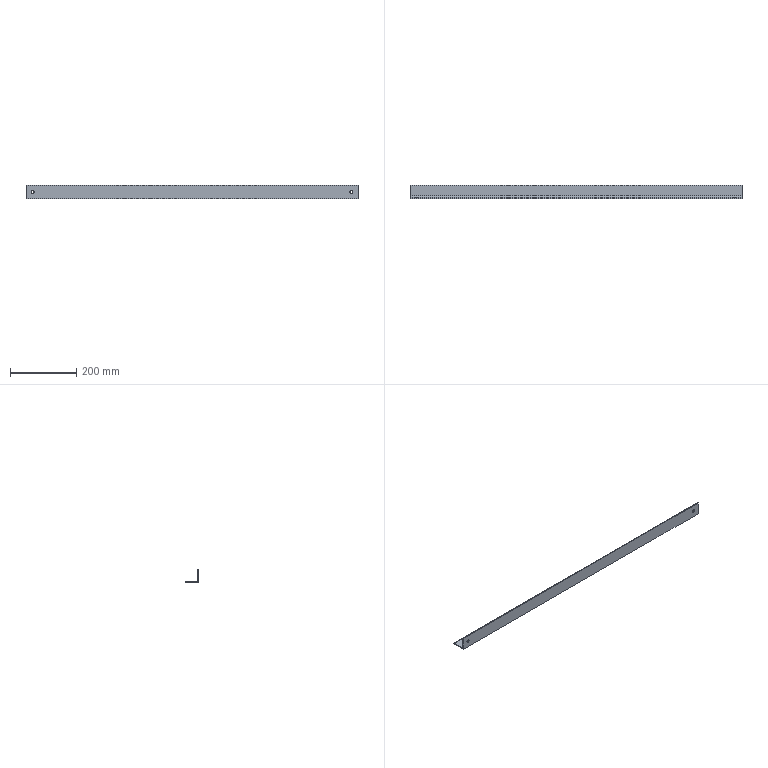Component | SolidWorks | SupportPlate-1 | 1 solid | 15 faces | box 1000 x 40 x 40 mm | volume 235554 mm3 | plane 8 | cylinder 7 | commonest cylinder face diameters 9 x4 2 x2 10 x1
build123d program:
from build123d import *

# Parameters (mm, degrees)
EQUAL_ANGLE_STEEL_40_X_40_X_3_1_DEPTH = 1000
SKETCH4_R                             = 4.5
CUT_EXTRUDE1_DEPTH                    = 504.19


with BuildPart() as part:
    # Sketch11 → Equal Angle Steel 40 X 40 X 3_1 (new body)
    with BuildSketch(Plane.YZ.offset(-500)):
        with BuildLine():
            Line((0, 0), (0, 40))
            Line((0, 40), (2, 40))
            ThreePointArc((2, 40), (2.707, 39.707), (3, 39))
            Line((3, 39), (3, 8))
            ThreePointArc((3, 8), (4.464, 4.464), (8, 3))
            Line((8, 3), (39, 3))
            ThreePointArc((39, 3), (39.707, 2.707), (40, 2))
            Line((40, 2), (40, 0))
            Line((40, 0), (0, 0))
        make_face()
    extrude(amount=EQUAL_ANGLE_STEEL_40_X_40_X_3_1_DEPTH)

    # Sketch4 → Cut-Extrude1 (cut, through all)
    with BuildSketch(Plane.XZ):
        with Locations(Location((-480, 20, 0), (0, 0, 270))):
            Circle(SKETCH4_R)
        with Locations(Location((480, 20, 0), (0, 0, 270))):
            Circle(SKETCH4_R)
    extrude(amount=-CUT_EXTRUDE1_DEPTH, mode=Mode.SUBTRACT)


solid = part.part

# Placed as in the assembly
solid = solid.moved(Location((434.468, -315.334, 1376.399), (0, 0, 0)))
STEP:
#1=COLOUR_RGB('',0.7922,0.8196,0.9333);
#2=FILL_AREA_STYLE_COLOUR('',#1);
#3=FILL_AREA_STYLE('',(#2));
#4=SURFACE_STYLE_FILL_AREA(#3);
#5=SURFACE_SIDE_STYLE('',(#4));
#6=SURFACE_STYLE_USAGE(.BOTH.,#5);
#7=PRESENTATION_STYLE_ASSIGNMENT((#6));
#8=CARTESIAN_POINT('',(36.003,-12.297,55.153));
#9=VERTEX_POINT('',#8);
#10=CARTESIAN_POINT('',(36.003,-12.297,54.799));
#11=VERTEX_POINT('',#10);
#12=CARTESIAN_POINT('',(36.003,-12.297,54.976));
#13=DIRECTION('',(0.,-1.,-0.));
#14=DIRECTION('',(0.,0.,-1.));
#15=AXIS2_PLACEMENT_3D('',#12,#13,#14);
#16=CIRCLE('',#15,0.1772);
#17=EDGE_CURVE('',#9,#11,#16,.T.);
#18=ORIENTED_EDGE('',*,*,#17,.F.);
#19=CARTESIAN_POINT('',(36.003,-12.415,55.153));
#20=VERTEX_POINT('',#19);
#21=CARTESIAN_POINT('',(36.003,-10.84,55.153));
#22=DIRECTION('',(0.,-1.,0.));
#23=VECTOR('',#22,39.37);
#24=LINE('',#21,#23);
#25=EDGE_CURVE('',#9,#20,#24,.T.);
#26=ORIENTED_EDGE('',*,*,#25,.T.);
#27=CARTESIAN_POINT('',(36.003,-12.415,54.799));
#28=VERTEX_POINT('',#27);
#29=CARTESIAN_POINT('',(36.003,-12.415,54.976));
#30=DIRECTION('',(0.,-1.,0.));
#31=DIRECTION('',(0.,0.,-1.));
#32=AXIS2_PLACEMENT_3D('',#29,#30,#31);
#33=CIRCLE('',#32,0.1772);
#34=EDGE_CURVE('',#20,#28,#33,.T.);
#35=ORIENTED_EDGE('',*,*,#34,.T.);
#36=CARTESIAN_POINT('',(36.003,-10.84,54.799));
#37=DIRECTION('',(0.,-1.,0.));
#38=VECTOR('',#37,39.37);
#39=LINE('',#36,#38);
#40=EDGE_CURVE('',#11,#28,#39,.T.);
#41=ORIENTED_EDGE('',*,*,#40,.F.);
#42=EDGE_LOOP('',(#18,#26,#35,#41));
#43=FACE_OUTER_BOUND('',#42,.T.);
#44=CARTESIAN_POINT('',(36.003,-10.84,54.976));
#45=DIRECTION('',(0.,-1.,0.));
#46=DIRECTION('',(0.,0.,-1.));
#47=AXIS2_PLACEMENT_3D('',#44,#45,#46);
#48=CYLINDRICAL_SURFACE('',#47,0.1772);
#49=ADVANCED_FACE('',(#43),#48,.F.);
#50=CARTESIAN_POINT('',(-1.793,-12.297,55.153));
#51=VERTEX_POINT('',#50);
#52=CARTESIAN_POINT('',(-1.793,-12.297,54.799));
#53=VERTEX_POINT('',#52);
#54=CARTESIAN_POINT('',(-1.793,-12.297,54.976));
#55=DIRECTION('',(0.,-1.,-0.));
#56=DIRECTION('',(0.,0.,-1.));
#57=AXIS2_PLACEMENT_3D('',#54,#55,#56);
#58=CIRCLE('',#57,0.1772);
#59=EDGE_CURVE('',#51,#53,#58,.T.);
#60=ORIENTED_EDGE('',*,*,#59,.F.);
#61=CARTESIAN_POINT('',(-1.793,-12.415,55.153));
#62=VERTEX_POINT('',#61);
#63=CARTESIAN_POINT('',(-1.793,-10.84,55.153));
#64=DIRECTION('',(0.,-1.,0.));
#65=VECTOR('',#64,39.37);
#66=LINE('',#63,#65);
#67=EDGE_CURVE('',#51,#62,#66,.T.);
#68=ORIENTED_EDGE('',*,*,#67,.T.);
#69=CARTESIAN_POINT('',(-1.793,-12.415,54.799));
#70=VERTEX_POINT('',#69);
#71=CARTESIAN_POINT('',(-1.793,-12.415,54.976));
#72=DIRECTION('',(0.,-1.,0.));
#73=DIRECTION('',(0.,0.,-1.));
#74=AXIS2_PLACEMENT_3D('',#71,#72,#73);
#75=CIRCLE('',#74,0.1772);
#76=EDGE_CURVE('',#62,#70,#75,.T.);
#77=ORIENTED_EDGE('',*,*,#76,.T.);
#78=CARTESIAN_POINT('',(-1.793,-10.84,54.799));
#79=DIRECTION('',(0.,-1.,0.));
#80=VECTOR('',#79,39.37);
#81=LINE('',#78,#80);
#82=EDGE_CURVE('',#53,#70,#81,.T.);
#83=ORIENTED_EDGE('',*,*,#82,.F.);
#84=EDGE_LOOP('',(#60,#68,#77,#83));
#85=FACE_OUTER_BOUND('',#84,.T.);
#86=CARTESIAN_POINT('',(-1.793,-10.84,54.976));
#87=DIRECTION('',(0.,-1.,0.));
#88=DIRECTION('',(0.,0.,-1.));
#89=AXIS2_PLACEMENT_3D('',#86,#87,#88);
#90=CYLINDRICAL_SURFACE('',#89,0.1772);
#91=ADVANCED_FACE('',(#85),#90,.F.);
#92=CARTESIAN_POINT('',(-2.58,-12.415,54.189));
#93=VERTEX_POINT('',#92);
#94=CARTESIAN_POINT('',(-2.58,-10.84,54.189));
#95=VERTEX_POINT('',#94);
#96=CARTESIAN_POINT('',(-2.58,-10.84,54.189));
#97=DIRECTION('',(0.,1.,0.));
#98=VECTOR('',#97,39.37);
#99=LINE('',#96,#98);
#100=EDGE_CURVE('',#93,#95,#99,.T.);
#101=ORIENTED_EDGE('',*,*,#100,.T.);
#102=CARTESIAN_POINT('',(36.79,-10.84,54.189));
#103=VERTEX_POINT('',#102);
#104=CARTESIAN_POINT('',(36.79,-10.84,54.189));
#105=DIRECTION('',(-1.,0.,0.));
#106=VECTOR('',#105,39.37);
#107=LINE('',#104,#106);
#108=EDGE_CURVE('',#103,#95,#107,.T.);
#109=ORIENTED_EDGE('',*,*,#108,.F.);
#110=CARTESIAN_POINT('',(36.79,-12.415,54.189));
#111=VERTEX_POINT('',#110);
#112=CARTESIAN_POINT('',(36.79,-10.84,54.189));
#113=DIRECTION('',(0.,1.,0.));
#114=VECTOR('',#113,39.37);
#115=LINE('',#112,#114);
#116=EDGE_CURVE('',#111,#103,#115,.T.);
#117=ORIENTED_EDGE('',*,*,#116,.F.);
#118=CARTESIAN_POINT('',(36.79,-12.415,54.189));
#119=DIRECTION('',(-1.,0.,0.));
#120=VECTOR('',#119,39.37);
#121=LINE('',#118,#120);
#122=EDGE_CURVE('',#111,#93,#121,.T.);
#123=ORIENTED_EDGE('',*,*,#122,.T.);
#124=EDGE_LOOP('',(#101,#109,#117,#123));
#125=FACE_OUTER_BOUND('',#124,.T.);
#126=CARTESIAN_POINT('',(36.79,-10.84,54.189));
#127=DIRECTION('',(0.,0.,1.));
#128=DIRECTION('',(1.,0.,0.));
#129=AXIS2_PLACEMENT_3D('',#126,#127,#128);
#130=PLANE('',#129);
#131=ADVANCED_FACE('',(#125),#130,.F.);
#132=CARTESIAN_POINT('',(-2.58,-10.84,54.268));
#133=VERTEX_POINT('',#132);
#134=CARTESIAN_POINT('',(-2.58,-10.84,54.189));
#135=DIRECTION('',(0.,0.,1.));
#136=VECTOR('',#135,39.37);
#137=LINE('',#134,#136);
#138=EDGE_CURVE('',#95,#133,#137,.T.);
#139=ORIENTED_EDGE('',*,*,#138,.T.);
#140=CARTESIAN_POINT('',(36.79,-10.84,54.268));
#141=VERTEX_POINT('',#140);
#142=CARTESIAN_POINT('',(36.79,-10.84,54.268));
#143=DIRECTION('',(-1.,0.,0.));
#144=VECTOR('',#143,39.37);
#145=LINE('',#142,#144);
#146=EDGE_CURVE('',#141,#133,#145,.T.);
#147=ORIENTED_EDGE('',*,*,#146,.F.);
#148=CARTESIAN_POINT('',(36.79,-10.84,54.189));
#149=DIRECTION('',(0.,0.,1.));
#150=VECTOR('',#149,39.37);
#151=LINE('',#148,#150);
#152=EDGE_CURVE('',#103,#141,#151,.T.);
#153=ORIENTED_EDGE('',*,*,#152,.F.);
#154=ORIENTED_EDGE('',*,*,#108,.T.);
#155=EDGE_LOOP('',(#139,#147,#153,#154));
#156=FACE_OUTER_BOUND('',#155,.T.);
#157=CARTESIAN_POINT('',(36.79,-10.84,54.189));
#158=DIRECTION('',(0.,-1.,0.));
#159=DIRECTION('',(0.,0.,-1.));
#160=AXIS2_PLACEMENT_3D('',#157,#158,#159);
#161=PLANE('',#160);
#162=ADVANCED_FACE('',(#156),#161,.F.);
#163=CARTESIAN_POINT('',(-2.58,-10.879,54.307));
#164=VERTEX_POINT('',#163);
#165=CARTESIAN_POINT('',(-2.58,-10.879,54.268));
#166=DIRECTION('',(1.,0.,0.));
#167=DIRECTION('',(0.,0.,-1.));
#168=AXIS2_PLACEMENT_3D('',#165,#166,#167);
#169=CIRCLE('',#168,0.03937);
#170=EDGE_CURVE('',#133,#164,#169,.T.);
#171=ORIENTED_EDGE('',*,*,#170,.T.);
#172=CARTESIAN_POINT('',(36.79,-10.879,54.307));
#173=VERTEX_POINT('',#172);
#174=CARTESIAN_POINT('',(36.79,-10.879,54.307));
#175=DIRECTION('',(-1.,0.,0.));
#176=VECTOR('',#175,39.37);
#177=LINE('',#174,#176);
#178=EDGE_CURVE('',#173,#164,#177,.T.);
#179=ORIENTED_EDGE('',*,*,#178,.F.);
#180=CARTESIAN_POINT('',(36.79,-10.879,54.268));
#181=DIRECTION('',(1.,0.,0.));
#182=DIRECTION('',(0.,0.,-1.));
#183=AXIS2_PLACEMENT_3D('',#180,#181,#182);
#184=CIRCLE('',#183,0.03937);
#185=EDGE_CURVE('',#141,#173,#184,.T.);
#186=ORIENTED_EDGE('',*,*,#185,.F.);
#187=ORIENTED_EDGE('',*,*,#146,.T.);
#188=EDGE_LOOP('',(#171,#179,#186,#187));
#189=FACE_OUTER_BOUND('',#188,.T.);
#190=CARTESIAN_POINT('',(36.79,-10.879,54.268));
#191=DIRECTION('',(-1.,0.,0.));
#192=DIRECTION('',(0.,0.,1.));
#193=AXIS2_PLACEMENT_3D('',#190,#191,#192);
#194=CYLINDRICAL_SURFACE('',#193,0.03937);
#195=ADVANCED_FACE('',(#189),#194,.T.);
#196=CARTESIAN_POINT('',(-2.58,-12.1,54.307));
#197=VERTEX_POINT('',#196);
#198=CARTESIAN_POINT('',(-2.58,-12.1,54.307));
#199=DIRECTION('',(0.,-1.,-0.));
#200=VECTOR('',#199,39.37);
#201=LINE('',#198,#200);
#202=EDGE_CURVE('',#164,#197,#201,.T.);
#203=ORIENTED_EDGE('',*,*,#202,.T.);
#204=CARTESIAN_POINT('',(36.79,-12.1,54.307));
#205=VERTEX_POINT('',#204);
#206=CARTESIAN_POINT('',(36.79,-12.1,54.307));
#207=DIRECTION('',(-1.,0.,0.));
#208=VECTOR('',#207,39.37);
#209=LINE('',#206,#208);
#210=EDGE_CURVE('',#205,#197,#209,.T.);
#211=ORIENTED_EDGE('',*,*,#210,.F.);
#212=CARTESIAN_POINT('',(36.79,-12.1,54.307));
#213=DIRECTION('',(0.,-1.,-0.));
#214=VECTOR('',#213,39.37);
#215=LINE('',#212,#214);
#216=EDGE_CURVE('',#173,#205,#215,.T.);
#217=ORIENTED_EDGE('',*,*,#216,.F.);
#218=ORIENTED_EDGE('',*,*,#178,.T.);
#219=EDGE_LOOP('',(#203,#211,#217,#218));
#220=FACE_OUTER_BOUND('',#219,.T.);
#221=CARTESIAN_POINT('',(36.79,-12.1,54.307));
#222=DIRECTION('',(0.,0.,-1.));
#223=DIRECTION('',(0.,1.,0.));
#224=AXIS2_PLACEMENT_3D('',#221,#222,#223);
#225=PLANE('',#224);
#226=ADVANCED_FACE('',(#220),#225,.F.);
#227=CARTESIAN_POINT('',(-2.58,-12.297,54.504));
#228=VERTEX_POINT('',#227);
#229=CARTESIAN_POINT('',(-2.58,-12.1,54.504));
#230=DIRECTION('',(-1.,0.,0.));
#231=DIRECTION('',(0.,0.,1.));
#232=AXIS2_PLACEMENT_3D('',#229,#230,#231);
#233=CIRCLE('',#232,0.1969);
#234=EDGE_CURVE('',#197,#228,#233,.T.);
#235=ORIENTED_EDGE('',*,*,#234,.T.);
#236=CARTESIAN_POINT('',(36.79,-12.297,54.504));
#237=VERTEX_POINT('',#236);
#238=CARTESIAN_POINT('',(36.79,-12.297,54.504));
#239=DIRECTION('',(-1.,0.,0.));
#240=VECTOR('',#239,39.37);
#241=LINE('',#238,#240);
#242=EDGE_CURVE('',#237,#228,#241,.T.);
#243=ORIENTED_EDGE('',*,*,#242,.F.);
#244=CARTESIAN_POINT('',(36.79,-12.1,54.504));
#245=DIRECTION('',(-1.,0.,0.));
#246=DIRECTION('',(0.,0.,1.));
#247=AXIS2_PLACEMENT_3D('',#244,#245,#246);
#248=CIRCLE('',#247,0.1969);
#249=EDGE_CURVE('',#205,#237,#248,.T.);
#250=ORIENTED_EDGE('',*,*,#249,.F.);
#251=ORIENTED_EDGE('',*,*,#210,.T.);
#252=EDGE_LOOP('',(#235,#243,#250,#251));
#253=FACE_OUTER_BOUND('',#252,.T.);
#254=CARTESIAN_POINT('',(36.79,-12.1,54.504));
#255=DIRECTION('',(-1.,0.,0.));
#256=DIRECTION('',(0.,0.,1.));
#257=AXIS2_PLACEMENT_3D('',#254,#255,#256);
#258=CYLINDRICAL_SURFACE('',#257,0.1969);
#259=ADVANCED_FACE('',(#253),#258,.F.);
#260=CARTESIAN_POINT('',(36.003,-12.297,54.976));
#261=DIRECTION('',(0.,-1.,-0.));
#262=DIRECTION('',(0.,0.,-1.));
#263=AXIS2_PLACEMENT_3D('',#260,#261,#262);
#264=CIRCLE('',#263,0.1772);
#265=EDGE_CURVE('',#11,#9,#264,.T.);
#266=ORIENTED_EDGE('',*,*,#265,.T.);
#267=ORIENTED_EDGE('',*,*,#17,.T.);
#268=EDGE_LOOP('',(#266,#267));
#269=FACE_BOUND('',#268,.T.);
#270=CARTESIAN_POINT('',(-1.793,-12.297,54.976));
#271=DIRECTION('',(0.,-1.,-0.));
#272=DIRECTION('',(0.,0.,-1.));
#273=AXIS2_PLACEMENT_3D('',#270,#271,#272);
#274=CIRCLE('',#273,0.1772);
#275=EDGE_CURVE('',#53,#51,#274,.T.);
#276=ORIENTED_EDGE('',*,*,#275,.T.);
#277=ORIENTED_EDGE('',*,*,#59,.T.);
#278=EDGE_LOOP('',(#276,#277));
#279=FACE_BOUND('',#278,.T.);
#280=CARTESIAN_POINT('',(-2.58,-12.297,55.724));
#281=VERTEX_POINT('',#280);
#282=CARTESIAN_POINT('',(-2.58,-12.297,55.724));
#283=DIRECTION('',(0.,-0.,1.));
#284=VECTOR('',#283,39.37);
#285=LINE('',#282,#284);
#286=EDGE_CURVE('',#228,#281,#285,.T.);
#287=ORIENTED_EDGE('',*,*,#286,.T.);
#288=CARTESIAN_POINT('',(36.79,-12.297,55.724));
#289=VERTEX_POINT('',#288);
#290=CARTESIAN_POINT('',(36.79,-12.297,55.724));
#291=DIRECTION('',(-1.,0.,0.));
#292=VECTOR('',#291,39.37);
#293=LINE('',#290,#292);
#294=EDGE_CURVE('',#289,#281,#293,.T.);
#295=ORIENTED_EDGE('',*,*,#294,.F.);
#296=CARTESIAN_POINT('',(36.79,-12.297,55.724));
#297=DIRECTION('',(0.,-0.,1.));
#298=VECTOR('',#297,39.37);
#299=LINE('',#296,#298);
#300=EDGE_CURVE('',#237,#289,#299,.T.);
#301=ORIENTED_EDGE('',*,*,#300,.F.);
#302=ORIENTED_EDGE('',*,*,#242,.T.);
#303=EDGE_LOOP('',(#287,#295,#301,#302));
#304=FACE_OUTER_BOUND('',#303,.T.);
#305=CARTESIAN_POINT('',(36.79,-12.297,55.724));
#306=DIRECTION('',(0.,-1.,-0.));
#307=DIRECTION('',(0.,0.,-1.));
#308=AXIS2_PLACEMENT_3D('',#305,#306,#307);
#309=PLANE('',#308);
#310=ADVANCED_FACE('',(#269,#279,#304),#309,.F.);
#311=CARTESIAN_POINT('',(-2.58,-12.336,55.764));
#312=VERTEX_POINT('',#311);
#313=CARTESIAN_POINT('',(-2.58,-12.336,55.724));
#314=DIRECTION('',(1.,0.,0.));
#315=DIRECTION('',(0.,0.,1.));
#316=AXIS2_PLACEMENT_3D('',#313,#314,#315);
#317=CIRCLE('',#316,0.03937);
#318=EDGE_CURVE('',#281,#312,#317,.T.);
#319=ORIENTED_EDGE('',*,*,#318,.T.);
#320=CARTESIAN_POINT('',(36.79,-12.336,55.764));
#321=VERTEX_POINT('',#320);
#322=CARTESIAN_POINT('',(36.79,-12.336,55.764));
#323=DIRECTION('',(-1.,0.,0.));
#324=VECTOR('',#323,39.37);
#325=LINE('',#322,#324);
#326=EDGE_CURVE('',#321,#312,#325,.T.);
#327=ORIENTED_EDGE('',*,*,#326,.F.);
#328=CARTESIAN_POINT('',(36.79,-12.336,55.724));
#329=DIRECTION('',(1.,0.,0.));
#330=DIRECTION('',(0.,0.,1.));
#331=AXIS2_PLACEMENT_3D('',#328,#329,#330);
#332=CIRCLE('',#331,0.03937);
#333=EDGE_CURVE('',#289,#321,#332,.T.);
#334=ORIENTED_EDGE('',*,*,#333,.F.);
#335=ORIENTED_EDGE('',*,*,#294,.T.);
#336=EDGE_LOOP('',(#319,#327,#334,#335));
#337=FACE_OUTER_BOUND('',#336,.T.);
#338=CARTESIAN_POINT('',(36.79,-12.336,55.724));
#339=DIRECTION('',(-1.,0.,0.));
#340=DIRECTION('',(0.,0.,1.));
#341=AXIS2_PLACEMENT_3D('',#338,#339,#340);
#342=CYLINDRICAL_SURFACE('',#341,0.03937);
#343=ADVANCED_FACE('',(#337),#342,.T.);
#344=CARTESIAN_POINT('',(-2.58,-12.415,55.764));
#345=VERTEX_POINT('',#344);
#346=CARTESIAN_POINT('',(-2.58,-12.415,55.764));
#347=DIRECTION('',(0.,-1.,0.));
#348=VECTOR('',#347,39.37);
#349=LINE('',#346,#348);
#350=EDGE_CURVE('',#312,#345,#349,.T.);
#351=ORIENTED_EDGE('',*,*,#350,.T.);
#352=CARTESIAN_POINT('',(36.79,-12.415,55.764));
#353=VERTEX_POINT('',#352);
#354=CARTESIAN_POINT('',(36.79,-12.415,55.764));
#355=DIRECTION('',(-1.,0.,0.));
#356=VECTOR('',#355,39.37);
#357=LINE('',#354,#356);
#358=EDGE_CURVE('',#353,#345,#357,.T.);
#359=ORIENTED_EDGE('',*,*,#358,.F.);
#360=CARTESIAN_POINT('',(36.79,-12.415,55.764));
#361=DIRECTION('',(0.,-1.,0.));
#362=VECTOR('',#361,39.37);
#363=LINE('',#360,#362);
#364=EDGE_CURVE('',#321,#353,#363,.T.);
#365=ORIENTED_EDGE('',*,*,#364,.F.);
#366=ORIENTED_EDGE('',*,*,#326,.T.);
#367=EDGE_LOOP('',(#351,#359,#365,#366));
#368=FACE_OUTER_BOUND('',#367,.T.);
#369=CARTESIAN_POINT('',(36.79,-12.415,55.764));
#370=DIRECTION('',(0.,0.,-1.));
#371=DIRECTION('',(-1.,0.,0.));
#372=AXIS2_PLACEMENT_3D('',#369,#370,#371);
#373=PLANE('',#372);
#374=ADVANCED_FACE('',(#368),#373,.F.);
#375=CARTESIAN_POINT('',(36.003,-12.415,54.976));
#376=DIRECTION('',(0.,-1.,0.));
#377=DIRECTION('',(0.,0.,-1.));
#378=AXIS2_PLACEMENT_3D('',#375,#376,#377);
#379=CIRCLE('',#378,0.1772);
#380=EDGE_CURVE('',#28,#20,#379,.T.);
#381=ORIENTED_EDGE('',*,*,#380,.F.);
#382=ORIENTED_EDGE('',*,*,#34,.F.);
#383=EDGE_LOOP('',(#381,#382));
#384=FACE_BOUND('',#383,.T.);
#385=CARTESIAN_POINT('',(-1.793,-12.415,54.976));
#386=DIRECTION('',(0.,-1.,0.));
#387=DIRECTION('',(0.,0.,-1.));
#388=AXIS2_PLACEMENT_3D('',#385,#386,#387);
#389=CIRCLE('',#388,0.1772);
#390=EDGE_CURVE('',#70,#62,#389,.T.);
#391=ORIENTED_EDGE('',*,*,#390,.F.);
#392=ORIENTED_EDGE('',*,*,#76,.F.);
#393=EDGE_LOOP('',(#391,#392));
#394=FACE_BOUND('',#393,.T.);
#395=CARTESIAN_POINT('',(-2.58,-12.415,54.189));
#396=DIRECTION('',(0.,0.,-1.));
#397=VECTOR('',#396,39.37);
#398=LINE('',#395,#397);
#399=EDGE_CURVE('',#345,#93,#398,.T.);
#400=ORIENTED_EDGE('',*,*,#399,.T.);
#401=ORIENTED_EDGE('',*,*,#122,.F.);
#402=CARTESIAN_POINT('',(36.79,-12.415,54.189));
#403=DIRECTION('',(0.,0.,-1.));
#404=VECTOR('',#403,39.37);
#405=LINE('',#402,#404);
#406=EDGE_CURVE('',#353,#111,#405,.T.);
#407=ORIENTED_EDGE('',*,*,#406,.F.);
#408=ORIENTED_EDGE('',*,*,#358,.T.);
#409=EDGE_LOOP('',(#400,#401,#407,#408));
#410=FACE_OUTER_BOUND('',#409,.T.);
#411=CARTESIAN_POINT('',(36.79,-12.415,54.189));
#412=DIRECTION('',(0.,1.,0.));
#413=DIRECTION('',(0.,0.,1.));
#414=AXIS2_PLACEMENT_3D('',#411,#412,#413);
#415=PLANE('',#414);
#416=ADVANCED_FACE('',(#384,#394,#410),#415,.F.);
#417=ORIENTED_EDGE('',*,*,#116,.T.);
#418=ORIENTED_EDGE('',*,*,#152,.T.);
#419=ORIENTED_EDGE('',*,*,#185,.T.);
#420=ORIENTED_EDGE('',*,*,#216,.T.);
#421=ORIENTED_EDGE('',*,*,#249,.T.);
#422=ORIENTED_EDGE('',*,*,#300,.T.);
#423=ORIENTED_EDGE('',*,*,#333,.T.);
#424=ORIENTED_EDGE('',*,*,#364,.T.);
#425=ORIENTED_EDGE('',*,*,#406,.T.);
#426=EDGE_LOOP('',(#417,#418,#419,#420,#421,#422,#423,#424,#425));
#427=FACE_OUTER_BOUND('',#426,.T.);
#428=CARTESIAN_POINT('',(36.79,-12.336,55.724));
#429=DIRECTION('',(-1.,0.,0.));
#430=DIRECTION('',(0.,0.,1.));
#431=AXIS2_PLACEMENT_3D('',#428,#429,#430);
#432=PLANE('',#431);
#433=ADVANCED_FACE('',(#427),#432,.F.);
#434=ORIENTED_EDGE('',*,*,#100,.F.);
#435=ORIENTED_EDGE('',*,*,#399,.F.);
#436=ORIENTED_EDGE('',*,*,#350,.F.);
#437=ORIENTED_EDGE('',*,*,#318,.F.);
#438=ORIENTED_EDGE('',*,*,#286,.F.);
#439=ORIENTED_EDGE('',*,*,#234,.F.);
#440=ORIENTED_EDGE('',*,*,#202,.F.);
#441=ORIENTED_EDGE('',*,*,#170,.F.);
#442=ORIENTED_EDGE('',*,*,#138,.F.);
#443=EDGE_LOOP('',(#434,#435,#436,#437,#438,#439,#440,#441,#442));
#444=FACE_OUTER_BOUND('',#443,.T.);
#445=CARTESIAN_POINT('',(-2.58,-12.336,55.724));
#446=DIRECTION('',(-1.,0.,0.));
#447=DIRECTION('',(0.,0.,1.));
#448=AXIS2_PLACEMENT_3D('',#445,#446,#447);
#449=PLANE('',#448);
#450=ADVANCED_FACE('',(#444),#449,.T.);
#451=ORIENTED_EDGE('',*,*,#67,.F.);
#452=ORIENTED_EDGE('',*,*,#275,.F.);
#453=ORIENTED_EDGE('',*,*,#82,.T.);
#454=ORIENTED_EDGE('',*,*,#390,.T.);
#455=EDGE_LOOP('',(#451,#452,#453,#454));
#456=FACE_OUTER_BOUND('',#455,.T.);
#457=CARTESIAN_POINT('',(-1.793,-10.84,54.976));
#458=DIRECTION('',(0.,-1.,0.));
#459=DIRECTION('',(0.,0.,-1.));
#460=AXIS2_PLACEMENT_3D('',#457,#458,#459);
#461=CYLINDRICAL_SURFACE('',#460,0.1772);
#462=ADVANCED_FACE('',(#456),#461,.F.);
#463=ORIENTED_EDGE('',*,*,#25,.F.);
#464=ORIENTED_EDGE('',*,*,#265,.F.);
#465=ORIENTED_EDGE('',*,*,#40,.T.);
#466=ORIENTED_EDGE('',*,*,#380,.T.);
#467=EDGE_LOOP('',(#463,#464,#465,#466));
#468=FACE_OUTER_BOUND('',#467,.T.);
#469=CARTESIAN_POINT('',(36.003,-10.84,54.976));
#470=DIRECTION('',(0.,-1.,0.));
#471=DIRECTION('',(0.,0.,-1.));
#472=AXIS2_PLACEMENT_3D('',#469,#470,#471);
#473=CYLINDRICAL_SURFACE('',#472,0.1772);
#474=ADVANCED_FACE('',(#468),#473,.F.);
#475=CLOSED_SHELL('',(#49,#91,#131,#162,#195,#226,#259,#310,#343,#374,#416,#433,#450,#462,#474));
#476=MANIFOLD_SOLID_BREP('',#475);
#477=STYLED_ITEM('',(#7),#476);
#478=(LENGTH_UNIT()NAMED_UNIT(*)SI_UNIT($,.METRE.));
#479=LENGTH_MEASURE_WITH_UNIT(LENGTH_MEASURE(0.0254),#478);
#480=DIMENSIONAL_EXPONENTS(1.,0.,0.,0.,0.,0.,0.);
#481=(CONVERSION_BASED_UNIT('',#479)LENGTH_UNIT()NAMED_UNIT(#480));
#482=UNCERTAINTY_MEASURE_WITH_UNIT(LENGTH_MEASURE(0.00001),#481,'','');
#483=(NAMED_UNIT(*)PLANE_ANGLE_UNIT()SI_UNIT($,.RADIAN.));
#484=(NAMED_UNIT(*)SI_UNIT($,.STERADIAN.)SOLID_ANGLE_UNIT());
#485=(GEOMETRIC_REPRESENTATION_CONTEXT(3)GLOBAL_UNCERTAINTY_ASSIGNED_CONTEXT((#482))GLOBAL_UNIT_ASSIGNED_CONTEXT((#481,#483,#484))REPRESENTATION_CONTEXT('',''));
#486=MECHANICAL_DESIGN_GEOMETRIC_PRESENTATION_REPRESENTATION('',(#477),#485);
#487=CARTESIAN_POINT('',(0.,0.,0.));
#488=DIRECTION('',(0.,0.,1.));
#489=DIRECTION('',(1.,0.,0.));
#490=AXIS2_PLACEMENT_3D('',#487,#488,#489);
#491=(LENGTH_UNIT()NAMED_UNIT(*)SI_UNIT($,.METRE.));
#492=LENGTH_MEASURE_WITH_UNIT(LENGTH_MEASURE(0.0254),#491);
#493=DIMENSIONAL_EXPONENTS(1.,0.,0.,0.,0.,0.,0.);
#494=(CONVERSION_BASED_UNIT('',#492)LENGTH_UNIT()NAMED_UNIT(#493));
#495=UNCERTAINTY_MEASURE_WITH_UNIT(LENGTH_MEASURE(0.00001),#494,'','');
#496=(NAMED_UNIT(*)PLANE_ANGLE_UNIT()SI_UNIT($,.RADIAN.));
#497=(NAMED_UNIT(*)SI_UNIT($,.STERADIAN.)SOLID_ANGLE_UNIT());
#498=(GEOMETRIC_REPRESENTATION_CONTEXT(3)GLOBAL_UNCERTAINTY_ASSIGNED_CONTEXT((#495))GLOBAL_UNIT_ASSIGNED_CONTEXT((#494,#496,#497))REPRESENTATION_CONTEXT('',''));
#499=ADVANCED_BREP_SHAPE_REPRESENTATION('',(#476,#490),#498);
#500=PRESENTATION_LAYER_ASSIGNMENT('','',(#477));